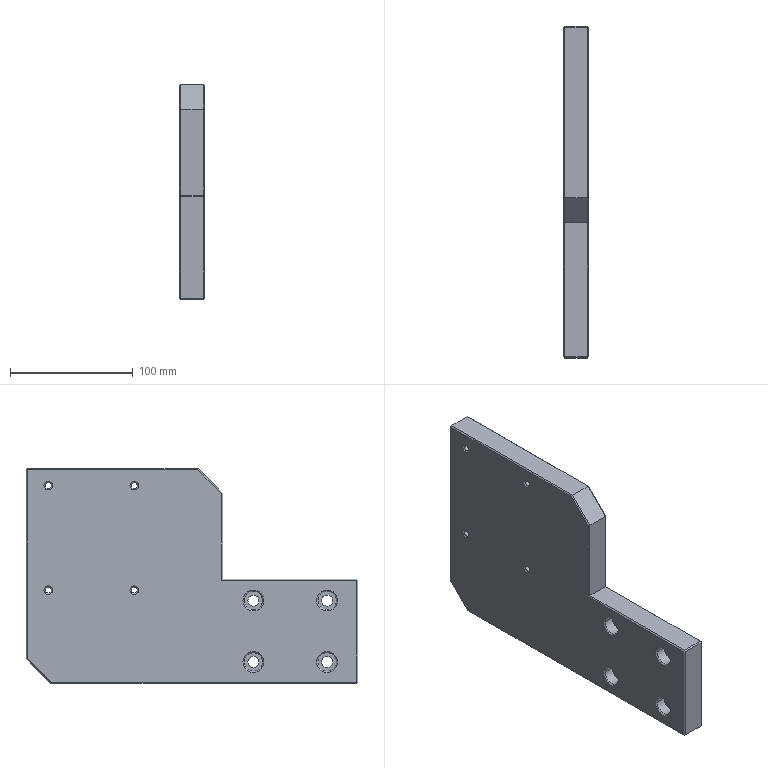Component | SolidWorks | CutterFixingPlateB-1 | 1 solid | 95 faces | box 20 x 270 x 175 mm | volume 727146 mm3 | plane 39 | cone 32 | cylinder 24 | commonest cylinder face diameters 15 x8 9 x8 5 x8 | material 1060 Alloy
build123d program:
from build123d import *

# Parameters (mm, degrees)
BOSS_EXTRUDE1_DEPTH                                = 20
M6_TAPPED_HOLE1_D                                  = 5
CHAMFER1_SIZE                                      = 20
SKETCH6_W                                          = 396.906
SKETCH6_H                                          = 363.651
CUT_EXTRUDE1_DEPTH                                 = 463.52
HOLE_SIZE_ACCORDING_TO_TYPE_OF_HEXAGON_D           = 9
HOLE_SIZE_ACCORDING_TO_TYPE_OF_HEXAGON_CBORE_D     = 15
HOLE_SIZE_ACCORDING_TO_TYPE_OF_HEXAGON_CBORE_DEPTH = 9
CHAMFER2_SIZE                                      = 1


with BuildPart() as part:
    # Sketch1 → Boss-Extrude1 (new body)
    with BuildSketch(Plane.XY):
        Polygon((0, 0), (0, 315), (60, 375), (270, 375), (270, 225), (100, 225), (100, 85), (270, 85), (270, -90), (110, -90), (110, 0), align=None)
    extrude(amount=BOSS_EXTRUDE1_DEPTH)

    # M6 Tapped Hole1 (through all)
    with Locations(Plane.XY.offset(20)):
        with Locations((182, 340), (252, 340), (252, 9), (182, 9), (182, 255), (252, 255), (252, -76), (182, -76)):
            Hole(M6_TAPPED_HOLE1_D / 2)

    # Chamfer1
    chamfer1_edges = [part.edges().sort_by_distance(p)[0] for p in [
        (270, 375, 10),
        (270, 225, 10),
        (100, 225, 10),
        (100, 85, 10),
        (270, 85, 10),
        (110, -90, 10),
    ]]
    chamfer(chamfer1_edges, length=CHAMFER1_SIZE)

    # Sketch6 → Cut-Extrude1 (cut, through all)
    with BuildSketch(Plane.XY.offset(20)):
        with Locations((144.544, 266.825)):
            Rectangle(SKETCH6_W, SKETCH6_H)
    extrude(amount=-CUT_EXTRUDE1_DEPTH, mode=Mode.SUBTRACT)

    # Hole Size _according to_ type of Hexagon (through all)
    with Locations(Plane.XY.offset(20)):
        with Locations((25, 67.5), (85, 67.5), (85, 17.5), (25, 17.5)):
            CounterBoreHole(HOLE_SIZE_ACCORDING_TO_TYPE_OF_HEXAGON_D / 2, HOLE_SIZE_ACCORDING_TO_TYPE_OF_HEXAGON_CBORE_D / 2, HOLE_SIZE_ACCORDING_TO_TYPE_OF_HEXAGON_CBORE_DEPTH)

    # Chamfer2
    chamfer2_edges = [part.edges().sort_by_distance(p)[0] for p in [
        (0, 42.5, 0),
        (0, 42.5, 20),
        (0, 85, 10),
        (270, -12.5, 0),
        (270, -12.5, 20),
        (110, -35, 0),
        (55, 0, 0),
        (17.5, 17.5, 20),
        (29.5, 17.5, 0),
        (77.5, 17.5, 20),
        (89.5, 17.5, 0),
        (77.5, 67.5, 20),
        (89.5, 67.5, 0),
        (0, 0, 10),
        (17.5, 67.5, 20),
        (29.5, 67.5, 0),
        (270, -90, 10),
        (184.5, -76, 20),
        (184.5, -76, 0),
        (55, 0, 20),
        (254.5, -76, 20),
        (254.5, -76, 0),
        (184.5, 9, 20),
        (184.5, 9, 0),
        (254.5, 9, 20),
        (254.5, 9, 0),
        (110, -35, 20),
        (200, -90, 0),
        (200, -90, 20),
        (125, 85, 0),
        (260, 75, 0),
        (120, -80, 0),
        (125, 85, 20),
        (260, 75, 20),
        (120, -80, 20),
    ]]
    chamfer(chamfer2_edges, length=CHAMFER2_SIZE)


solid = part.part

# Placed as in the assembly
solid = solid.moved(Location((-144.666, 130.264, 197.5), (-90, -90, 0)))